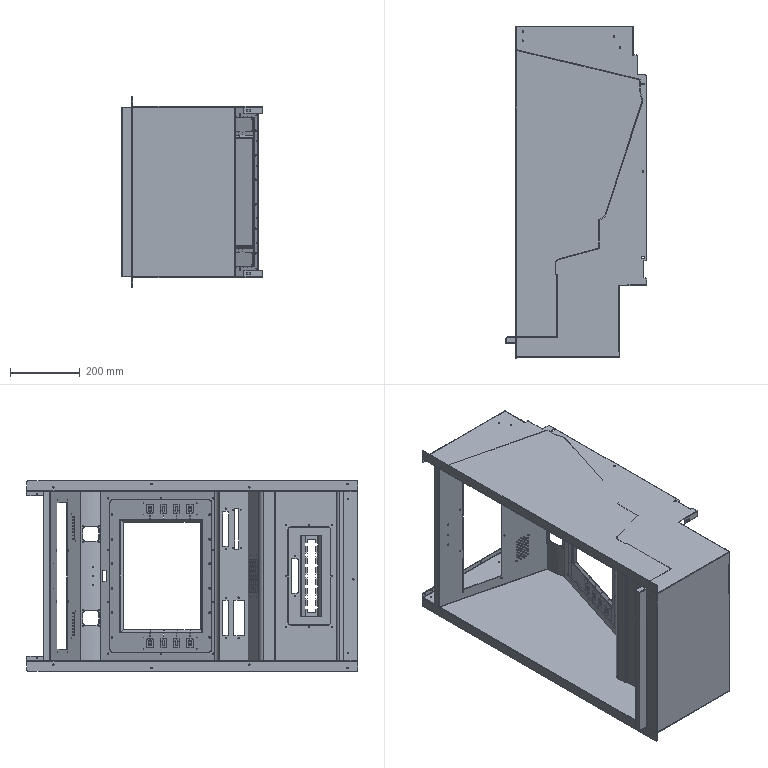Assembly | SolidWorks | mm | 16 component files | 16 solids | 2302 faces | box 403 x 947.9 x 545 mm | volume 3408698 mm3 | plane 1268 | cylinder 837 | spline 197 | commonest cylinder face diameters 2.5 x242 4 x196 5 x77 4.4 x48 0.4 x48 5.5 x36 6 x30 4.05 x22
Bill of materials:
BottomPlate | 1 |  | Bent thin-sheet panel: a large flat rectangular web with a short return flange along one long edge and an offset narrow tab along the opposite edge, giving a stepped/Z-like section.
DisplayPanel | 1 |  | Flat rectangular frame plate with rounded outer corners and a large central rectangular opening. The opening edge has a short bent lip with relief cuts, there is a row of four rectangular slots above and below the opening, and small holes run around the perimeter.
NavigationKey | 2 |  | Elongated rectangular box/bar-like body with four small holes near the corners of one long face. One view shows a strip with a series of small rectangular notches along one edge.
TouchScreenPanel | 1 |  | Very thin flat rectangular frame (gasket- or shim-like ring of material) with a large rectangular opening, many small holes around the border, and a shallow rectangular notch in one outer side edge.
Keyboard | 1 |  | Square slab- or shallow-box-like body with noticeable thickness. Small rectangular notches are spaced along two adjacent edges.
LeftSidePlate | 1 |  | Long flat sheet plate with a bent flange along one long edge and short partial flanges on the opposite edge. That edge has a stepped outline with notches and tabs, and there are scattered small holes.
Panel | 1 |  | Large multi-bend sheet panel folded into several faceted segments, giving an open stepped profile. It has several large rectangular openings, smaller rectangular slots, patches of small perforations and many small perimeter holes.
RightSidePlate | 1 |  | Long flat sheet plate with a stepped outline, small holes and bent edge flanges. It is close in shape to unnamed part, but its flanges appear to turn in the opposite direction.
CashDispenserGasket | 1 |  | Thin flat rectangular frame with rounded outer corners and a large rectangular opening with small inner corner radii. It has eight round holes: one at each corner and one at the middle of each side.
CashDispenserNozzle | 1 |  | Long bent sheet channel/post with an open section: an angled leg, a straight web and a curved leg, joined by rounded bends. The web has a long central slot with evenly spaced rectangular notches along both sides.
CashDispenserNozzleSidePlate | 2 |  | Flat plate with an irregular four-sided outline: straight edges, one concave curved edge and rounded corners. It has no holes and is moderately thick compared with the sheet parts.
CashDispenserPanel | 1 |  | Thin flat rectangular plate with rounded corners, a large rectangular opening on one side, and a smaller rounded-corner rectangular slot beside it with a small hole above and below the slot.
PlacketLeftHangerPlate | 1 |  | Thin, uniform-thickness formed plate (looks like bent sheet) with an irregular outline: a long straight edge, a long angled taper edge, and a stepped rectangular tab at the narrow end. Flanges are bent downward along several edges with small inside bend radii. One end flange folds back underneath into a C-shaped return lip.
PlacketRightHangerPlate | 1 |  | Thin formed plate with nearly the same outline as the other part: straight long edge, angled taper edge, stepped rectangular tab. Here the flanges at the wide end are bent upward, forming a shallow tray-like corner. A flange along the tab side is bent downward and has a small round hole. The narrow end has a C-shaped return lip with a curved hook-like cutout.
Mates:
1. coincident | Panel-1 face at (-42.033, -507.058, 242.5) dir (1, 0, 0) | YarnOutletAssembly-2/CashDispenserGasket-1 face at (-42.033, -496.058, -147) dir (-1, 0, 0)
2. concentric | Panel-1 face at (74.967, -362.058, -145) dir (-1, 0, 0) r 2 | YarnOutletAssembly-2/CashDispenserGasket-1 face at (-42.033, -362.058, -145) dir (1, 0, 0) r 2.75
3. concentric | Panel-1 face at (74.967, -494.058, -145) dir (-1, 0, 0) r 2 | YarnOutletAssembly-2/CashDispenserGasket-1 face at (-42.033, -494.058, -145) dir (1, 0, 0) r 2.75
4. coincident | Panel-1 face at (-189.033, -515.058, 242.5) dir (1, 0, 0) | BottomPlate-1 face at (-189.033, -509.058, -242.5) dir (-1, 0, 0)
5. coincident | Panel-1 face at (-183.033, -509.058, -242.5) dir (0, 0, -1) | BottomPlate-1 face at (-161.233, -509.058, -242.5) dir (0, 0, -1)
6. concentric | Panel-1 face at (-183.033, -515.058, 485.112) dir (0, 0, -1) r 6 | BottomPlate-1 face at (-183.033, -515.058, -242.5) dir (0, 0, 1) r 6
7. coincident | Panel-1 face at (-189.033, -515.058, 242.5) dir (0, 0, 1) | LeftSidePlate-1 face at (182.067, 295.942, 242.5) dir (0, 0, -1)
8. coincident | Panel-1 face at (-161.033, 331.579, 242.5) dir (-1, 0, 0) | LeftSidePlate-1 face at (-161.033, -567.058, 244.5) dir (-1, 0, 0)
9. coincident | BottomPlate-1 face at (135.467, -567.058, 242.5) dir (0, -1, 0) | LeftSidePlate-1 face at (135.467, -567.058, 244.5) dir (0, -1, 0)
10. distance | Keyboard-1 face at (60.262, -259.933, -46) dir (0, 0, -1) | Panel-1 face at (62.574, -267.596, -46.25) dir (0, 0, 1)
11. distance | Keyboard-1 face at (60.262, -259.933, -46) dir (0.9659, 0.2588, 0) | Panel-1 face at (62.574, -267.596, 46.25) dir (-0.9659, -0.2588, 0)
12. distance | Keyboard-1 face at (16.019, -268.682, -44.54) dir (-0.2588, 0.9659, 0) | Panel-1 face at (-37.915, -284.169, 242.5) dir (-0.2588, 0.9659, 0)
13. coincident | Panel-1 face at (95.89, -157.721, 242.5) dir (0.9511, -0.309, 0) | DisplayPanel-1/TouchScreenPanel-1 face at (194.331, 145.248, 222.5) dir (-0.9511, 0.309, 0)
14. concentric | Panel-1 face at (104.445, -157.282, -222) dir (-0.9511, 0.309, 0) r 2 | DisplayPanel-1/TouchScreenPanel-1 face at (96.836, -154.81, -222) dir (0.9511, -0.309, 0) r 2.75
15. concentric | Panel-1 face at (104.445, -157.282, -74) dir (-0.9511, 0.309, 0) r 2 | DisplayPanel-1/TouchScreenPanel-1 face at (96.836, -154.81, -74) dir (0.9511, -0.309, 0) r 2.75
16. coincident | DisplayPanel-1 face at (-272.248, 126.008, 2.096) dir (0, 0, -1) | TouchScreenPanel-1 face at (168.052, 130.708, 2.096) dir (0, 0, 1)
17. concentric | DisplayPanel-1 face at (120.552, -173.792, 2.096) dir (0, 0, 1) r 2.5 | TouchScreenPanel-1 face at (120.552, -173.792, 2.096) dir (0, 0, -1) r 2.5
18. concentric | DisplayPanel-1 face at (-229.448, -173.792, 2.096) dir (0, 0, 1) r 2.5 | TouchScreenPanel-1 face at (-229.448, -173.792, 2.096) dir (0, 0, -1) r 2.5
19. concentric | DisplayPanel-1 face at (-230.198, 25.458, 2.096) dir (0, 0, 1) r 1.058 | NavigationKey-1 face at (-230.198, 25.458, 2.096) dir (0, 0, -1) r 1.25
20. coincident | DisplayPanel-1 face at (-272.248, 126.008, 2.096) dir (0, 0, -1) | NavigationKey-1 face at (-226.198, -143.792, 2.096) dir (0, 0, 1)
21. concentric | DisplayPanel-1 face at (-230.198, -134.542, 2.096) dir (0, 0, 1) r 1.058 | NavigationKey-1 face at (-230.198, -134.542, 2.096) dir (0, 0, -1) r 1.25
22. concentric | DisplayPanel-1 face at (121.302, 25.458, 2.096) dir (0, 0, 1) r 1.058 | NavigationKey-2 face at (121.302, 25.458, 2.096) dir (0, 0, -1) r 1.25
23. concentric | DisplayPanel-1 face at (153.802, 25.458, 2.096) dir (0, 0, 1) r 1.058 | NavigationKey-2 face at (153.802, 25.458, 2.096) dir (0, 0, -1) r 1.25
24. coincident | DisplayPanel-1 face at (-272.248, 126.008, 2.096) dir (0, 0, -1) | NavigationKey-2 face at (117.302, 34.708, 2.096) dir (0, 0, 1)
25. coincident | CashDispenserGasket-1 face at (-132.12, 51.532, -1) dir (0, 0, -1) | CashDispenserPanel-1 face at (147.38, 36.532, -1) dir (0, 0, 1)
26. distance | CashDispenserPanel-1 face at (147.38, -76.968, -3) dir (0, -1, 0) | CashDispenserGasket-1 face at (-132.12, -87.468, -1) dir (0, -1, 0)
27. distance | CashDispenserPanel-1 face at (-125.12, 36.532, -3) dir (-1, 0, 0) | CashDispenserGasket-1 face at (-135.12, 51.532, -1) dir (-1, 0, 0)
28. concentric | CashDispenserNozzle-1 face at (-102.12, 47.321, 22.919) dir (1, 0, 0) r 40 | CashDispenserNozzleSidePlate-1 face at (-104.12, 47.321, 22.919) dir (1, 0, 0) r 38
29. parallel | CashDispenserNozzle-1 face at (-102.12, -27.827, 20) dir (0, 0, -1) | CashDispenserNozzleSidePlate-1 face at (-104.12, -27.696, 22) dir (0, 0, 1)
30. coincident | CashDispenserNozzle-1 face at (-102.12, 9.479, 19.455) dir (-1, 0, 0) | CashDispenserNozzleSidePlate-1 face at (-102.12, -27.696, 19) dir (1, 0, 0)
31. coincident | CashDispenserNozzle-1 face at (131.88, 7.488, 19.273) dir (1, 0, 0) | CashDispenserNozzleSidePlate-2 face at (131.88, -27.696, 19) dir (-1, 0, 0)
32. coincident | CashDispenserNozzle-1 face at (-102.12, -27.827, 22) dir (0, 0, 1) | CashDispenserNozzleSidePlate-2 face at (131.88, -27.696, 22) dir (0, 0, 1)
33. coincident | CashDispenserNozzle-1 face at (-102.12, -30.398, 20.31) dir (0, -0.918, 0.3966) | CashDispenserNozzleSidePlate-2 face at (131.88, -39.604, -1) dir (0, -0.918, 0.3966)
34. coincident | CashDispenserPanel-1 face at (147.38, 36.532, -1) dir (0, 0, 1) | CashDispenserNozzleSidePlate-2 face at (131.88, 17.793, -1) dir (0, 0, -1)
35. coincident | CashDispenserPanel-1 face at (-102.12, 19.532, -3) dir (1, 0, 0) | CashDispenserNozzle-1 face at (-102.12, -27.827, 20) dir (-1, 0, 0)
36. coincident | CashDispenserPanel-1 edge at (-102.12, -40.468, -3) dir (1, 0, 0) | CashDispenserNozzle-1 edge at (-102.12, -40.468, -3) dir (1, 0, 0)
37. coincident | CashDispenserPanel-1 face at (147.38, 36.532, -1) dir (0, 0, 1) | PlacketRightHangerPlate-1 face at (-114.42, -58.968, -1) dir (0, 0, -1)
38. distance | PlacketRightHangerPlate-1 face at (-116.62, 32.032, 26) dir (-1, 0, 0) | CashDispenserGasket-1 face at (-135.12, 51.532, -1) dir (-1, 0, 0)
39. distance | PlacketRightHangerPlate-1 face at (-104.62, -60.968, 24) dir (0, -1, 0) | CashDispenserGasket-1 face at (-132.12, -87.468, -1) dir (0, -1, 0)